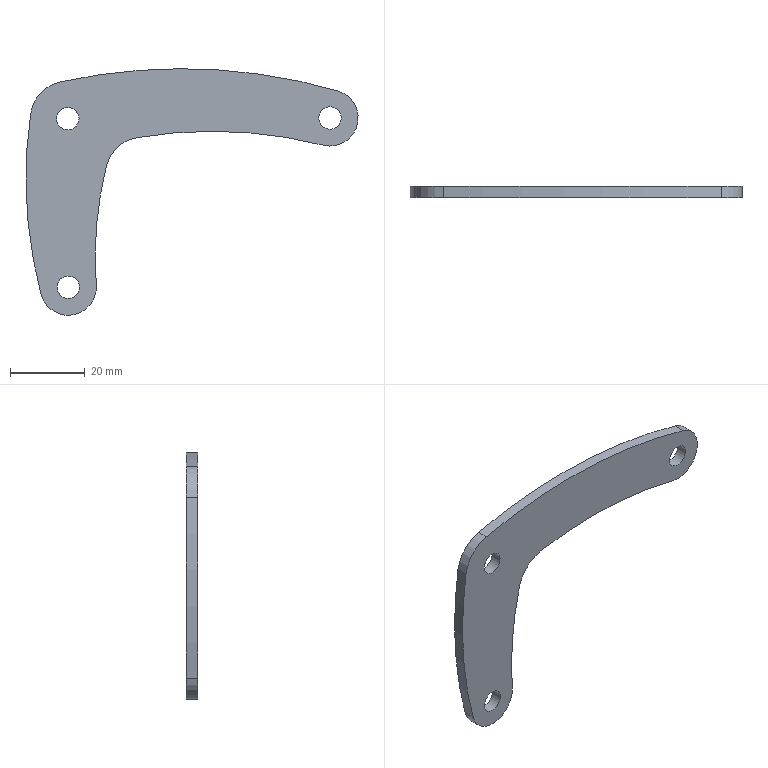Component | NX | LINK_2_3 | 1 solid | 13 faces | box 88.67 x 3 x 65.83 mm | volume 6437 mm3 | cylinder 11 | plane 2 | commonest cylinder face diameters 6 x3 240 x2 20 x2 15 x2 300 x1 200 x1
STEP:
#1=CARTESIAN_POINT('',(0.,0.,0.));
#2=DIRECTION('',(0.,0.,1.));
#3=DIRECTION('',(1.,0.,0.));
#4=AXIS2_PLACEMENT_3D('',#1,#2,#3);
#5=CARTESIAN_POINT('',(-172.247,90.,70.568));
#6=VERTEX_POINT('',#5);
#7=CARTESIAN_POINT('',(-175.02,90.,118.956));
#8=VERTEX_POINT('',#7);
#9=CARTESIAN_POINT('',(-56.298,90.,101.486));
#10=DIRECTION('',(0.,1.,0.));
#11=DIRECTION('',(-1.,0.,-0.002813));
#12=AXIS2_PLACEMENT_3D('',#9,#10,#11);
#13=CIRCLE('',#12,120.);
#14=CARTESIAN_POINT('',(-56.298,93.,101.486));
#15=DIRECTION('',(0.,-1.,0.));
#16=DIRECTION('',(-0.002813,0.,1.));
#17=AXIS2_PLACEMENT_3D('',#14,#15,#16);
#18=CYLINDRICAL_SURFACE('',#17,120.);
#19=CARTESIAN_POINT('',(7.854,3.));
#20=DIRECTION('',(-1.,0.));
#21=VECTOR('',#20,1.);
#22=LINE('',#19,#21);
#23=(GEOMETRIC_REPRESENTATION_CONTEXT(2)PARAMETRIC_REPRESENTATION_CONTEXT()REPRESENTATION_CONTEXT('',''));
#24=DEFINITIONAL_REPRESENTATION('',(#22),#23);
#25=PCURVE('',#18,#24);
#26=CARTESIAN_POINT('',(-110.713,90.,109.493));
#27=DIRECTION('',(0.,1.,0.));
#28=DIRECTION('',(0.002813,0.,-1.));
#29=AXIS2_PLACEMENT_3D('',#26,#27,#28);
#30=PLANE('',#29);
#31=CARTESIAN_POINT('',(8.16,-54.391));
#32=DIRECTION('',(0.,1.));
#33=AXIS2_PLACEMENT_2D('',#31,#32);
#34=CIRCLE('',#33,120.);
#35=(GEOMETRIC_REPRESENTATION_CONTEXT(2)PARAMETRIC_REPRESENTATION_CONTEXT()REPRESENTATION_CONTEXT('',''));
#36=DEFINITIONAL_REPRESENTATION('',(#34),#35);
#37=PCURVE('',#30,#36);
#38=SURFACE_CURVE('',#13,(#25,#37),.PCURVE_S1.);
#39=EDGE_CURVE('',#6,#8,#38,.T.);
#40=ORIENTED_EDGE('',*,*,#39,.T.);
#41=CARTESIAN_POINT('',(-175.02,93.,118.956));
#42=VERTEX_POINT('',#41);
#43=CARTESIAN_POINT('',(-175.02,93.,118.956));
#44=DIRECTION('',(0.,-1.,0.));
#45=VECTOR('',#44,1.);
#46=LINE('',#43,#45);
#47=CARTESIAN_POINT('',(1.422,0.));
#48=DIRECTION('',(0.,1.));
#49=VECTOR('',#48,1.);
#50=LINE('',#47,#49);
#51=(GEOMETRIC_REPRESENTATION_CONTEXT(2)PARAMETRIC_REPRESENTATION_CONTEXT()REPRESENTATION_CONTEXT('',''));
#52=DEFINITIONAL_REPRESENTATION('',(#50),#51);
#53=PCURVE('',#18,#52);
#54=CARTESIAN_POINT('',(-165.127,93.,117.5));
#55=DIRECTION('',(0.,-1.,0.));
#56=DIRECTION('',(-0.002813,0.,1.));
#57=AXIS2_PLACEMENT_3D('',#54,#55,#56);
#58=CYLINDRICAL_SURFACE('',#57,10.);
#59=CARTESIAN_POINT('',(1.422,0.));
#60=DIRECTION('',(0.,1.));
#61=VECTOR('',#60,1.);
#62=LINE('',#59,#61);
#63=(GEOMETRIC_REPRESENTATION_CONTEXT(2)PARAMETRIC_REPRESENTATION_CONTEXT()REPRESENTATION_CONTEXT('',''));
#64=DEFINITIONAL_REPRESENTATION('',(#62),#63);
#65=PCURVE('',#58,#64);
#66=SURFACE_CURVE('',#46,(#53,#65),.PCURVE_S1.);
#67=EDGE_CURVE('',#42,#8,#66,.T.);
#68=ORIENTED_EDGE('',*,*,#67,.F.);
#69=CARTESIAN_POINT('',(-172.247,93.,70.568));
#70=VERTEX_POINT('',#69);
#71=CARTESIAN_POINT('',(-56.298,93.,101.486));
#72=DIRECTION('',(0.,1.,0.));
#73=DIRECTION('',(-1.,0.,-0.002813));
#74=AXIS2_PLACEMENT_3D('',#71,#72,#73);
#75=CIRCLE('',#74,120.);
#76=CARTESIAN_POINT('',(7.854,0.));
#77=DIRECTION('',(-1.,0.));
#78=VECTOR('',#77,1.);
#79=LINE('',#76,#78);
#80=(GEOMETRIC_REPRESENTATION_CONTEXT(2)PARAMETRIC_REPRESENTATION_CONTEXT()REPRESENTATION_CONTEXT('',''));
#81=DEFINITIONAL_REPRESENTATION('',(#79),#80);
#82=PCURVE('',#18,#81);
#83=CARTESIAN_POINT('',(-110.713,93.,109.493));
#84=DIRECTION('',(0.,1.,0.));
#85=DIRECTION('',(0.002813,0.,-1.));
#86=AXIS2_PLACEMENT_3D('',#83,#84,#85);
#87=PLANE('',#86);
#88=CARTESIAN_POINT('',(8.16,-54.391));
#89=DIRECTION('',(0.,1.));
#90=AXIS2_PLACEMENT_2D('',#88,#89);
#91=CIRCLE('',#90,120.);
#92=(GEOMETRIC_REPRESENTATION_CONTEXT(2)PARAMETRIC_REPRESENTATION_CONTEXT()REPRESENTATION_CONTEXT('',''));
#93=DEFINITIONAL_REPRESENTATION('',(#91),#92);
#94=PCURVE('',#87,#93);
#95=SURFACE_CURVE('',#75,(#82,#94),.PCURVE_S1.);
#96=EDGE_CURVE('',#70,#42,#95,.T.);
#97=ORIENTED_EDGE('',*,*,#96,.F.);
#98=CARTESIAN_POINT('',(-172.247,93.,70.568));
#99=DIRECTION('',(0.,-1.,0.));
#100=VECTOR('',#99,1.);
#101=LINE('',#98,#100);
#102=CARTESIAN_POINT('',(1.829,0.));
#103=DIRECTION('',(0.,1.));
#104=VECTOR('',#103,1.);
#105=LINE('',#102,#104);
#106=(GEOMETRIC_REPRESENTATION_CONTEXT(2)PARAMETRIC_REPRESENTATION_CONTEXT()REPRESENTATION_CONTEXT('',''));
#107=DEFINITIONAL_REPRESENTATION('',(#105),#106);
#108=PCURVE('',#18,#107);
#109=CARTESIAN_POINT('',(-165.,93.,72.5));
#110=DIRECTION('',(0.,-1.,0.));
#111=DIRECTION('',(-0.002813,0.,1.));
#112=AXIS2_PLACEMENT_3D('',#109,#110,#111);
#113=CYLINDRICAL_SURFACE('',#112,7.5);
#114=CARTESIAN_POINT('',(1.829,0.));
#115=DIRECTION('',(0.,1.));
#116=VECTOR('',#115,1.);
#117=LINE('',#114,#116);
#118=(GEOMETRIC_REPRESENTATION_CONTEXT(2)PARAMETRIC_REPRESENTATION_CONTEXT()REPRESENTATION_CONTEXT('',''));
#119=DEFINITIONAL_REPRESENTATION('',(#117),#118);
#120=PCURVE('',#113,#119);
#121=SURFACE_CURVE('',#101,(#108,#120),.PCURVE_S1.);
#122=EDGE_CURVE('',#70,#6,#121,.T.);
#123=ORIENTED_EDGE('',*,*,#122,.T.);
#124=EDGE_LOOP('',(#40,#68,#97,#123));
#125=FACE_BOUND('',#124,.T.);
#126=ADVANCED_FACE('',(#125),#18,.T.);
#127=CARTESIAN_POINT('',(-167.294,90.,127.262));
#128=VERTEX_POINT('',#127);
#129=CARTESIAN_POINT('',(-165.127,90.,117.5));
#130=DIRECTION('',(0.,1.,0.));
#131=DIRECTION('',(-1.,0.,-0.002813));
#132=AXIS2_PLACEMENT_3D('',#129,#130,#131);
#133=CIRCLE('',#132,10.);
#134=CARTESIAN_POINT('',(1.571,3.));
#135=DIRECTION('',(-1.,0.));
#136=VECTOR('',#135,1.);
#137=LINE('',#134,#136);
#138=(GEOMETRIC_REPRESENTATION_CONTEXT(2)PARAMETRIC_REPRESENTATION_CONTEXT()REPRESENTATION_CONTEXT('',''));
#139=DEFINITIONAL_REPRESENTATION('',(#137),#138);
#140=PCURVE('',#58,#139);
#141=CARTESIAN_POINT('',(-8.16,54.391));
#142=DIRECTION('',(0.,1.));
#143=AXIS2_PLACEMENT_2D('',#141,#142);
#144=CIRCLE('',#143,10.);
#145=(GEOMETRIC_REPRESENTATION_CONTEXT(2)PARAMETRIC_REPRESENTATION_CONTEXT()REPRESENTATION_CONTEXT('',''));
#146=DEFINITIONAL_REPRESENTATION('',(#144),#145);
#147=PCURVE('',#30,#146);
#148=SURFACE_CURVE('',#133,(#140,#147),.PCURVE_S1.);
#149=EDGE_CURVE('',#8,#128,#148,.T.);
#150=ORIENTED_EDGE('',*,*,#149,.T.);
#151=CARTESIAN_POINT('',(-167.294,93.,127.262));
#152=VERTEX_POINT('',#151);
#153=CARTESIAN_POINT('',(-167.294,93.,127.262));
#154=DIRECTION('',(0.,-1.,0.));
#155=VECTOR('',#154,1.);
#156=LINE('',#153,#155);
#157=CARTESIAN_POINT('',(0.2156,0.));
#158=DIRECTION('',(0.,1.));
#159=VECTOR('',#158,1.);
#160=LINE('',#157,#159);
#161=(GEOMETRIC_REPRESENTATION_CONTEXT(2)PARAMETRIC_REPRESENTATION_CONTEXT()REPRESENTATION_CONTEXT('',''));
#162=DEFINITIONAL_REPRESENTATION('',(#160),#161);
#163=PCURVE('',#58,#162);
#164=CARTESIAN_POINT('',(-134.787,93.,-19.173));
#165=DIRECTION('',(0.,-1.,0.));
#166=DIRECTION('',(-0.002813,0.,1.));
#167=AXIS2_PLACEMENT_3D('',#164,#165,#166);
#168=CYLINDRICAL_SURFACE('',#167,150.);
#169=CARTESIAN_POINT('',(6.499,0.));
#170=DIRECTION('',(0.,1.));
#171=VECTOR('',#170,1.);
#172=LINE('',#169,#171);
#173=(GEOMETRIC_REPRESENTATION_CONTEXT(2)PARAMETRIC_REPRESENTATION_CONTEXT()REPRESENTATION_CONTEXT('',''));
#174=DEFINITIONAL_REPRESENTATION('',(#172),#173);
#175=PCURVE('',#168,#174);
#176=SURFACE_CURVE('',#156,(#163,#175),.PCURVE_S1.);
#177=EDGE_CURVE('',#152,#128,#176,.T.);
#178=ORIENTED_EDGE('',*,*,#177,.F.);
#179=CARTESIAN_POINT('',(-165.127,93.,117.5));
#180=DIRECTION('',(0.,1.,0.));
#181=DIRECTION('',(-1.,0.,-0.002813));
#182=AXIS2_PLACEMENT_3D('',#179,#180,#181);
#183=CIRCLE('',#182,10.);
#184=CARTESIAN_POINT('',(1.571,0.));
#185=DIRECTION('',(-1.,0.));
#186=VECTOR('',#185,1.);
#187=LINE('',#184,#186);
#188=(GEOMETRIC_REPRESENTATION_CONTEXT(2)PARAMETRIC_REPRESENTATION_CONTEXT()REPRESENTATION_CONTEXT('',''));
#189=DEFINITIONAL_REPRESENTATION('',(#187),#188);
#190=PCURVE('',#58,#189);
#191=CARTESIAN_POINT('',(-8.16,54.391));
#192=DIRECTION('',(0.,1.));
#193=AXIS2_PLACEMENT_2D('',#191,#192);
#194=CIRCLE('',#193,10.);
#195=(GEOMETRIC_REPRESENTATION_CONTEXT(2)PARAMETRIC_REPRESENTATION_CONTEXT()REPRESENTATION_CONTEXT('',''));
#196=DEFINITIONAL_REPRESENTATION('',(#194),#195);
#197=PCURVE('',#87,#196);
#198=SURFACE_CURVE('',#183,(#190,#197),.PCURVE_S1.);
#199=EDGE_CURVE('',#42,#152,#198,.T.);
#200=ORIENTED_EDGE('',*,*,#199,.F.);
#201=ORIENTED_EDGE('',*,*,#67,.T.);
#202=EDGE_LOOP('',(#150,#178,#200,#201));
#203=FACE_BOUND('',#202,.T.);
#204=ADVANCED_FACE('',(#203),#58,.T.);
#205=CARTESIAN_POINT('',(-93.04,90.,124.9));
#206=VERTEX_POINT('',#205);
#207=CARTESIAN_POINT('',(-134.787,90.,-19.173));
#208=DIRECTION('',(0.,1.,0.));
#209=DIRECTION('',(-1.,0.,-0.002813));
#210=AXIS2_PLACEMENT_3D('',#207,#208,#209);
#211=CIRCLE('',#210,150.);
#212=CARTESIAN_POINT('',(7.854,3.));
#213=DIRECTION('',(-1.,0.));
#214=VECTOR('',#213,1.);
#215=LINE('',#212,#214);
#216=(GEOMETRIC_REPRESENTATION_CONTEXT(2)PARAMETRIC_REPRESENTATION_CONTEXT()REPRESENTATION_CONTEXT('',''));
#217=DEFINITIONAL_REPRESENTATION('',(#215),#216);
#218=PCURVE('',#168,#217);
#219=CARTESIAN_POINT('',(128.598,24.436));
#220=DIRECTION('',(0.,1.));
#221=AXIS2_PLACEMENT_2D('',#219,#220);
#222=CIRCLE('',#221,150.);
#223=(GEOMETRIC_REPRESENTATION_CONTEXT(2)PARAMETRIC_REPRESENTATION_CONTEXT()REPRESENTATION_CONTEXT('',''));
#224=DEFINITIONAL_REPRESENTATION('',(#222),#223);
#225=PCURVE('',#30,#224);
#226=SURFACE_CURVE('',#211,(#218,#225),.PCURVE_S1.);
#227=EDGE_CURVE('',#128,#206,#226,.T.);
#228=ORIENTED_EDGE('',*,*,#227,.T.);
#229=CARTESIAN_POINT('',(-93.04,93.,124.9));
#230=VERTEX_POINT('',#229);
#231=CARTESIAN_POINT('',(-93.04,93.,124.9));
#232=DIRECTION('',(0.,-1.,0.));
#233=VECTOR('',#232,1.);
#234=LINE('',#231,#233);
#235=CARTESIAN_POINT('',(5.998,0.));
#236=DIRECTION('',(0.,1.));
#237=VECTOR('',#236,1.);
#238=LINE('',#235,#237);
#239=(GEOMETRIC_REPRESENTATION_CONTEXT(2)PARAMETRIC_REPRESENTATION_CONTEXT()REPRESENTATION_CONTEXT('',''));
#240=DEFINITIONAL_REPRESENTATION('',(#238),#239);
#241=PCURVE('',#168,#240);
#242=CARTESIAN_POINT('',(-95.127,93.,117.697));
#243=DIRECTION('',(0.,-1.,0.));
#244=DIRECTION('',(-0.002813,0.,1.));
#245=AXIS2_PLACEMENT_3D('',#242,#243,#244);
#246=CYLINDRICAL_SURFACE('',#245,7.5);
#247=CARTESIAN_POINT('',(5.998,0.));
#248=DIRECTION('',(0.,1.));
#249=VECTOR('',#248,1.);
#250=LINE('',#247,#249);
#251=(GEOMETRIC_REPRESENTATION_CONTEXT(2)PARAMETRIC_REPRESENTATION_CONTEXT()REPRESENTATION_CONTEXT('',''));
#252=DEFINITIONAL_REPRESENTATION('',(#250),#251);
#253=PCURVE('',#246,#252);
#254=SURFACE_CURVE('',#234,(#241,#253),.PCURVE_S1.);
#255=EDGE_CURVE('',#230,#206,#254,.T.);
#256=ORIENTED_EDGE('',*,*,#255,.F.);
#257=CARTESIAN_POINT('',(-134.787,93.,-19.173));
#258=DIRECTION('',(0.,1.,0.));
#259=DIRECTION('',(-1.,0.,-0.002813));
#260=AXIS2_PLACEMENT_3D('',#257,#258,#259);
#261=CIRCLE('',#260,150.);
#262=CARTESIAN_POINT('',(7.854,0.));
#263=DIRECTION('',(-1.,0.));
#264=VECTOR('',#263,1.);
#265=LINE('',#262,#264);
#266=(GEOMETRIC_REPRESENTATION_CONTEXT(2)PARAMETRIC_REPRESENTATION_CONTEXT()REPRESENTATION_CONTEXT('',''));
#267=DEFINITIONAL_REPRESENTATION('',(#265),#266);
#268=PCURVE('',#168,#267);
#269=CARTESIAN_POINT('',(128.598,24.436));
#270=DIRECTION('',(0.,1.));
#271=AXIS2_PLACEMENT_2D('',#269,#270);
#272=CIRCLE('',#271,150.);
#273=(GEOMETRIC_REPRESENTATION_CONTEXT(2)PARAMETRIC_REPRESENTATION_CONTEXT()REPRESENTATION_CONTEXT('',''));
#274=DEFINITIONAL_REPRESENTATION('',(#272),#273);
#275=PCURVE('',#87,#274);
#276=SURFACE_CURVE('',#261,(#268,#275),.PCURVE_S1.);
#277=EDGE_CURVE('',#152,#230,#276,.T.);
#278=ORIENTED_EDGE('',*,*,#277,.F.);
#279=ORIENTED_EDGE('',*,*,#177,.T.);
#280=EDGE_LOOP('',(#228,#256,#278,#279));
#281=FACE_BOUND('',#280,.T.);
#282=ADVANCED_FACE('',(#281),#168,.T.);
#283=CARTESIAN_POINT('',(-96.975,90.,110.428));
#284=VERTEX_POINT('',#283);
#285=CARTESIAN_POINT('',(-95.127,90.,117.697));
#286=DIRECTION('',(0.,1.,0.));
#287=DIRECTION('',(-1.,0.,-0.002813));
#288=AXIS2_PLACEMENT_3D('',#285,#286,#287);
#289=CIRCLE('',#288,7.5);
#290=CARTESIAN_POINT('',(7.854,3.));
#291=DIRECTION('',(-1.,0.));
#292=VECTOR('',#291,1.);
#293=LINE('',#290,#292);
#294=(GEOMETRIC_REPRESENTATION_CONTEXT(2)PARAMETRIC_REPRESENTATION_CONTEXT()REPRESENTATION_CONTEXT('',''));
#295=DEFINITIONAL_REPRESENTATION('',(#293),#294);
#296=PCURVE('',#246,#295);
#297=CARTESIAN_POINT('',(-8.16,-15.609));
#298=DIRECTION('',(-0.,1.));
#299=AXIS2_PLACEMENT_2D('',#297,#298);
#300=CIRCLE('',#299,7.5);
#301=(GEOMETRIC_REPRESENTATION_CONTEXT(2)PARAMETRIC_REPRESENTATION_CONTEXT()REPRESENTATION_CONTEXT('',''));
#302=DEFINITIONAL_REPRESENTATION('',(#300),#301);
#303=PCURVE('',#30,#302);
#304=SURFACE_CURVE('',#289,(#296,#303),.PCURVE_S1.);
#305=EDGE_CURVE('',#206,#284,#304,.T.);
#306=ORIENTED_EDGE('',*,*,#305,.T.);
#307=CARTESIAN_POINT('',(-96.975,93.,110.428));
#308=VERTEX_POINT('',#307);
#309=CARTESIAN_POINT('',(-96.975,93.,110.428));
#310=DIRECTION('',(0.,-1.,0.));
#311=VECTOR('',#310,1.);
#312=LINE('',#309,#311);
#313=CARTESIAN_POINT('',(2.89,0.));
#314=DIRECTION('',(0.,1.));
#315=VECTOR('',#314,1.);
#316=LINE('',#313,#315);
#317=(GEOMETRIC_REPRESENTATION_CONTEXT(2)PARAMETRIC_REPRESENTATION_CONTEXT()REPRESENTATION_CONTEXT('',''));
#318=DEFINITIONAL_REPRESENTATION('',(#316),#317);
#319=PCURVE('',#246,#318);
#320=CARTESIAN_POINT('',(-126.548,93.,-5.871));
#321=DIRECTION('',(0.,-1.,0.));
#322=DIRECTION('',(-0.002813,0.,1.));
#323=AXIS2_PLACEMENT_3D('',#320,#321,#322);
#324=CYLINDRICAL_SURFACE('',#323,120.);
#325=CARTESIAN_POINT('',(6.031,0.));
#326=DIRECTION('',(0.,1.));
#327=VECTOR('',#326,1.);
#328=LINE('',#325,#327);
#329=(GEOMETRIC_REPRESENTATION_CONTEXT(2)PARAMETRIC_REPRESENTATION_CONTEXT()REPRESENTATION_CONTEXT('',''));
#330=DEFINITIONAL_REPRESENTATION('',(#328),#329);
#331=PCURVE('',#324,#330);
#332=SURFACE_CURVE('',#312,(#319,#331),.PCURVE_S1.);
#333=EDGE_CURVE('',#308,#284,#332,.T.);
#334=ORIENTED_EDGE('',*,*,#333,.F.);
#335=CARTESIAN_POINT('',(-95.127,93.,117.697));
#336=DIRECTION('',(0.,1.,0.));
#337=DIRECTION('',(-1.,0.,-0.002813));
#338=AXIS2_PLACEMENT_3D('',#335,#336,#337);
#339=CIRCLE('',#338,7.5);
#340=CARTESIAN_POINT('',(7.854,0.));
#341=DIRECTION('',(-1.,0.));
#342=VECTOR('',#341,1.);
#343=LINE('',#340,#342);
#344=(GEOMETRIC_REPRESENTATION_CONTEXT(2)PARAMETRIC_REPRESENTATION_CONTEXT()REPRESENTATION_CONTEXT('',''));
#345=DEFINITIONAL_REPRESENTATION('',(#343),#344);
#346=PCURVE('',#246,#345);
#347=CARTESIAN_POINT('',(-8.16,-15.609));
#348=DIRECTION('',(-0.,1.));
#349=AXIS2_PLACEMENT_2D('',#347,#348);
#350=CIRCLE('',#349,7.5);
#351=(GEOMETRIC_REPRESENTATION_CONTEXT(2)PARAMETRIC_REPRESENTATION_CONTEXT()REPRESENTATION_CONTEXT('',''));
#352=DEFINITIONAL_REPRESENTATION('',(#350),#351);
#353=PCURVE('',#87,#352);
#354=SURFACE_CURVE('',#339,(#346,#353),.PCURVE_S1.);
#355=EDGE_CURVE('',#230,#308,#354,.T.);
#356=ORIENTED_EDGE('',*,*,#355,.F.);
#357=ORIENTED_EDGE('',*,*,#255,.T.);
#358=EDGE_LOOP('',(#306,#334,#356,#357));
#359=FACE_BOUND('',#358,.T.);
#360=ADVANCED_FACE('',(#359),#246,.T.);
#361=ORIENTED_EDGE('',*,*,#333,.F.);
#362=CARTESIAN_POINT('',(-146.77,93.,112.413));
#363=VERTEX_POINT('',#362);
#364=CARTESIAN_POINT('',(-126.548,93.,-5.871));
#365=DIRECTION('',(0.,-1.,0.));
#366=DIRECTION('',(-1.,0.,-0.002813));
#367=AXIS2_PLACEMENT_3D('',#364,#365,#366);
#368=CIRCLE('',#367,120.);
#369=CARTESIAN_POINT('',(1.571,0.));
#370=DIRECTION('',(1.,0.));
#371=VECTOR('',#370,1.);
#372=LINE('',#369,#371);
#373=(GEOMETRIC_REPRESENTATION_CONTEXT(2)PARAMETRIC_REPRESENTATION_CONTEXT()REPRESENTATION_CONTEXT('',''));
#374=DEFINITIONAL_REPRESENTATION('',(#372),#373);
#375=PCURVE('',#324,#374);
#376=CARTESIAN_POINT('',(115.319,136.16));
#377=CARTESIAN_POINT('',(323.165,136.16));
#378=CARTESIAN_POINT('',(219.242,-43.84));
#379=CARTESIAN_POINT('',(115.319,-223.84));
#380=CARTESIAN_POINT('',(11.396,-43.84));
#381=CARTESIAN_POINT('',(-92.527,136.16));
#382=CARTESIAN_POINT('',(115.319,136.16));
#383=(BOUNDED_CURVE()B_SPLINE_CURVE(2,(#376,#377,#378,#379,#380,#381,#382),.UNSPECIFIED.,.T.,.F.)B_SPLINE_CURVE_WITH_KNOTS((1,2,2,2,2,1),(-2.094,0.,2.094,4.189,6.283,8.378),.UNSPECIFIED.)CURVE()GEOMETRIC_REPRESENTATION_ITEM()RATIONAL_B_SPLINE_CURVE((1.,0.5,1.,0.5,1.,0.5,1.))REPRESENTATION_ITEM(''));
#384=(GEOMETRIC_REPRESENTATION_CONTEXT(2)PARAMETRIC_REPRESENTATION_CONTEXT()REPRESENTATION_CONTEXT('',''));
#385=DEFINITIONAL_REPRESENTATION('',(#383),#384);
#386=PCURVE('',#87,#385);
#387=SURFACE_CURVE('',#368,(#375,#386),.PCURVE_S1.);
#388=EDGE_CURVE('',#308,#363,#387,.T.);
#389=ORIENTED_EDGE('',*,*,#388,.T.);
#390=CARTESIAN_POINT('',(-146.77,90.,112.413));
#391=VERTEX_POINT('',#390);
#392=CARTESIAN_POINT('',(-146.77,93.,112.413));
#393=DIRECTION('',(0.,-1.,0.));
#394=VECTOR('',#393,1.);
#395=LINE('',#392,#394);
#396=CARTESIAN_POINT('',(6.45,0.));
#397=DIRECTION('',(0.,1.));
#398=VECTOR('',#397,1.);
#399=LINE('',#396,#398);
#400=(GEOMETRIC_REPRESENTATION_CONTEXT(2)PARAMETRIC_REPRESENTATION_CONTEXT()REPRESENTATION_CONTEXT('',''));
#401=DEFINITIONAL_REPRESENTATION('',(#399),#400);
#402=PCURVE('',#324,#401);
#403=CARTESIAN_POINT('',(-145.084,93.,102.556));
#404=DIRECTION('',(0.,-1.,0.));
#405=DIRECTION('',(-0.002813,0.,1.));
#406=AXIS2_PLACEMENT_3D('',#403,#404,#405);
#407=CYLINDRICAL_SURFACE('',#406,10.);
#408=CARTESIAN_POINT('',(0.1665,0.));
#409=DIRECTION('',(0.,1.));
#410=VECTOR('',#409,1.);
#411=LINE('',#408,#410);
#412=(GEOMETRIC_REPRESENTATION_CONTEXT(2)PARAMETRIC_REPRESENTATION_CONTEXT()REPRESENTATION_CONTEXT('',''));
#413=DEFINITIONAL_REPRESENTATION('',(#411),#412);
#414=PCURVE('',#407,#413);
#415=SURFACE_CURVE('',#395,(#402,#414),.PCURVE_S1.);
#416=EDGE_CURVE('',#363,#391,#415,.T.);
#417=ORIENTED_EDGE('',*,*,#416,.T.);
#418=CARTESIAN_POINT('',(-126.548,90.,-5.871));
#419=DIRECTION('',(0.,-1.,0.));
#420=DIRECTION('',(-1.,0.,-0.002813));
#421=AXIS2_PLACEMENT_3D('',#418,#419,#420);
#422=CIRCLE('',#421,120.);
#423=CARTESIAN_POINT('',(1.571,3.));
#424=DIRECTION('',(1.,0.));
#425=VECTOR('',#424,1.);
#426=LINE('',#423,#425);
#427=(GEOMETRIC_REPRESENTATION_CONTEXT(2)PARAMETRIC_REPRESENTATION_CONTEXT()REPRESENTATION_CONTEXT('',''));
#428=DEFINITIONAL_REPRESENTATION('',(#426),#427);
#429=PCURVE('',#324,#428);
#430=CARTESIAN_POINT('',(115.319,136.16));
#431=CARTESIAN_POINT('',(323.165,136.16));
#432=CARTESIAN_POINT('',(219.242,-43.84));
#433=CARTESIAN_POINT('',(115.319,-223.84));
#434=CARTESIAN_POINT('',(11.396,-43.84));
#435=CARTESIAN_POINT('',(-92.527,136.16));
#436=CARTESIAN_POINT('',(115.319,136.16));
#437=(BOUNDED_CURVE()B_SPLINE_CURVE(2,(#430,#431,#432,#433,#434,#435,#436),.UNSPECIFIED.,.T.,.F.)B_SPLINE_CURVE_WITH_KNOTS((1,2,2,2,2,1),(-2.094,0.,2.094,4.189,6.283,8.378),.UNSPECIFIED.)CURVE()GEOMETRIC_REPRESENTATION_ITEM()RATIONAL_B_SPLINE_CURVE((1.,0.5,1.,0.5,1.,0.5,1.))REPRESENTATION_ITEM(''));
#438=(GEOMETRIC_REPRESENTATION_CONTEXT(2)PARAMETRIC_REPRESENTATION_CONTEXT()REPRESENTATION_CONTEXT('',''));
#439=DEFINITIONAL_REPRESENTATION('',(#437),#438);
#440=PCURVE('',#30,#439);
#441=SURFACE_CURVE('',#422,(#429,#440),.PCURVE_S1.);
#442=EDGE_CURVE('',#284,#391,#441,.T.);
#443=ORIENTED_EDGE('',*,*,#442,.F.);
#444=EDGE_LOOP('',(#361,#389,#417,#443));
#445=FACE_BOUND('',#444,.F.);
#446=ADVANCED_FACE('',(#445),#324,.F.);
#447=ORIENTED_EDGE('',*,*,#416,.F.);
#448=CARTESIAN_POINT('',(-154.782,93.,104.996));
#449=VERTEX_POINT('',#448);
#450=CARTESIAN_POINT('',(-145.084,93.,102.556));
#451=DIRECTION('',(0.,-1.,0.));
#452=DIRECTION('',(-1.,0.,-0.002813));
#453=AXIS2_PLACEMENT_3D('',#450,#451,#452);
#454=CIRCLE('',#453,10.);
#455=CARTESIAN_POINT('',(-4.712,0.));
#456=DIRECTION('',(1.,0.));
#457=VECTOR('',#456,1.);
#458=LINE('',#455,#457);
#459=(GEOMETRIC_REPRESENTATION_CONTEXT(2)PARAMETRIC_REPRESENTATION_CONTEXT()REPRESENTATION_CONTEXT('',''));
#460=DEFINITIONAL_REPRESENTATION('',(#458),#459);
#461=PCURVE('',#407,#460);
#462=CARTESIAN_POINT('',(6.84,44.391));
#463=CARTESIAN_POINT('',(24.161,44.391));
#464=CARTESIAN_POINT('',(15.501,29.391));
#465=CARTESIAN_POINT('',(6.84,14.391));
#466=CARTESIAN_POINT('',(-1.82,29.391));
#467=CARTESIAN_POINT('',(-10.48,44.391));
#468=CARTESIAN_POINT('',(6.84,44.391));
#469=(BOUNDED_CURVE()B_SPLINE_CURVE(2,(#462,#463,#464,#465,#466,#467,#468),.UNSPECIFIED.,.T.,.F.)B_SPLINE_CURVE_WITH_KNOTS((1,2,2,2,2,1),(-2.094,0.,2.094,4.189,6.283,8.378),.UNSPECIFIED.)CURVE()GEOMETRIC_REPRESENTATION_ITEM()RATIONAL_B_SPLINE_CURVE((1.,0.5,1.,0.5,1.,0.5,1.))REPRESENTATION_ITEM(''));
#470=(GEOMETRIC_REPRESENTATION_CONTEXT(2)PARAMETRIC_REPRESENTATION_CONTEXT()REPRESENTATION_CONTEXT('',''));
#471=DEFINITIONAL_REPRESENTATION('',(#469),#470);
#472=PCURVE('',#87,#471);
#473=SURFACE_CURVE('',#454,(#461,#472),.PCURVE_S1.);
#474=EDGE_CURVE('',#363,#449,#473,.T.);
#475=ORIENTED_EDGE('',*,*,#474,.T.);
#476=CARTESIAN_POINT('',(-154.782,90.,104.996));
#477=VERTEX_POINT('',#476);
#478=CARTESIAN_POINT('',(-154.782,93.,104.996));
#479=DIRECTION('',(0.,-1.,0.));
#480=VECTOR('',#479,1.);
#481=LINE('',#478,#480);
#482=CARTESIAN_POINT('',(1.321,0.));
#483=DIRECTION('',(0.,1.));
#484=VECTOR('',#483,1.);
#485=LINE('',#482,#484);
#486=(GEOMETRIC_REPRESENTATION_CONTEXT(2)PARAMETRIC_REPRESENTATION_CONTEXT()REPRESENTATION_CONTEXT('',''));
#487=DEFINITIONAL_REPRESENTATION('',(#485),#486);
#488=PCURVE('',#407,#487);
#489=CARTESIAN_POINT('',(-57.805,93.,80.594));
#490=DIRECTION('',(0.,-1.,0.));
#491=DIRECTION('',(-0.002813,0.,1.));
#492=AXIS2_PLACEMENT_3D('',#489,#490,#491);
#493=CYLINDRICAL_SURFACE('',#492,100.);
#494=CARTESIAN_POINT('',(1.321,0.));
#495=DIRECTION('',(0.,1.));
#496=VECTOR('',#495,1.);
#497=LINE('',#494,#496);
#498=(GEOMETRIC_REPRESENTATION_CONTEXT(2)PARAMETRIC_REPRESENTATION_CONTEXT()REPRESENTATION_CONTEXT('',''));
#499=DEFINITIONAL_REPRESENTATION('',(#497),#498);
#500=PCURVE('',#493,#499);
#501=SURFACE_CURVE('',#481,(#488,#500),.PCURVE_S1.);
#502=EDGE_CURVE('',#449,#477,#501,.T.);
#503=ORIENTED_EDGE('',*,*,#502,.T.);
#504=CARTESIAN_POINT('',(-145.084,90.,102.556));
#505=DIRECTION('',(0.,-1.,0.));
#506=DIRECTION('',(-1.,0.,-0.002813));
#507=AXIS2_PLACEMENT_3D('',#504,#505,#506);
#508=CIRCLE('',#507,10.);
#509=CARTESIAN_POINT('',(-4.712,3.));
#510=DIRECTION('',(1.,0.));
#511=VECTOR('',#510,1.);
#512=LINE('',#509,#511);
#513=(GEOMETRIC_REPRESENTATION_CONTEXT(2)PARAMETRIC_REPRESENTATION_CONTEXT()REPRESENTATION_CONTEXT('',''));
#514=DEFINITIONAL_REPRESENTATION('',(#512),#513);
#515=PCURVE('',#407,#514);
#516=CARTESIAN_POINT('',(6.84,44.391));
#517=CARTESIAN_POINT('',(24.161,44.391));
#518=CARTESIAN_POINT('',(15.501,29.391));
#519=CARTESIAN_POINT('',(6.84,14.391));
#520=CARTESIAN_POINT('',(-1.82,29.391));
#521=CARTESIAN_POINT('',(-10.48,44.391));
#522=CARTESIAN_POINT('',(6.84,44.391));
#523=(BOUNDED_CURVE()B_SPLINE_CURVE(2,(#516,#517,#518,#519,#520,#521,#522),.UNSPECIFIED.,.T.,.F.)B_SPLINE_CURVE_WITH_KNOTS((1,2,2,2,2,1),(-2.094,0.,2.094,4.189,6.283,8.378),.UNSPECIFIED.)CURVE()GEOMETRIC_REPRESENTATION_ITEM()RATIONAL_B_SPLINE_CURVE((1.,0.5,1.,0.5,1.,0.5,1.))REPRESENTATION_ITEM(''));
#524=(GEOMETRIC_REPRESENTATION_CONTEXT(2)PARAMETRIC_REPRESENTATION_CONTEXT()REPRESENTATION_CONTEXT('',''));
#525=DEFINITIONAL_REPRESENTATION('',(#523),#524);
#526=PCURVE('',#30,#525);
#527=SURFACE_CURVE('',#508,(#515,#526),.PCURVE_S1.);
#528=EDGE_CURVE('',#391,#477,#527,.T.);
#529=ORIENTED_EDGE('',*,*,#528,.F.);
#530=EDGE_LOOP('',(#447,#475,#503,#529));
#531=FACE_BOUND('',#530,.F.);
#532=ADVANCED_FACE('',(#531),#407,.F.);
#533=ORIENTED_EDGE('',*,*,#502,.F.);
#534=CARTESIAN_POINT('',(-157.521,93.,73.065));
#535=VERTEX_POINT('',#534);
#536=CARTESIAN_POINT('',(-57.805,93.,80.594));
#537=DIRECTION('',(0.,-1.,0.));
#538=DIRECTION('',(-1.,0.,-0.002813));
#539=AXIS2_PLACEMENT_3D('',#536,#537,#538);
#540=CIRCLE('',#539,100.);
#541=CARTESIAN_POINT('',(-4.712,0.));
#542=DIRECTION('',(1.,0.));
#543=VECTOR('',#542,1.);
#544=LINE('',#541,#543);
#545=(GEOMETRIC_REPRESENTATION_CONTEXT(2)PARAMETRIC_REPRESENTATION_CONTEXT()REPRESENTATION_CONTEXT('',''));
#546=DEFINITIONAL_REPRESENTATION('',(#544),#545);
#547=PCURVE('',#493,#546);
#548=CARTESIAN_POINT('',(29.048,47.174));
#549=CARTESIAN_POINT('',(202.253,47.174));
#550=CARTESIAN_POINT('',(115.65,-102.826));
#551=CARTESIAN_POINT('',(29.048,-252.826));
#552=CARTESIAN_POINT('',(-57.555,-102.826));
#553=CARTESIAN_POINT('',(-144.158,47.174));
#554=CARTESIAN_POINT('',(29.048,47.174));
#555=(BOUNDED_CURVE()B_SPLINE_CURVE(2,(#548,#549,#550,#551,#552,#553,#554),.UNSPECIFIED.,.T.,.F.)B_SPLINE_CURVE_WITH_KNOTS((1,2,2,2,2,1),(-2.094,0.,2.094,4.189,6.283,8.378),.UNSPECIFIED.)CURVE()GEOMETRIC_REPRESENTATION_ITEM()RATIONAL_B_SPLINE_CURVE((1.,0.5,1.,0.5,1.,0.5,1.))REPRESENTATION_ITEM(''));
#556=(GEOMETRIC_REPRESENTATION_CONTEXT(2)PARAMETRIC_REPRESENTATION_CONTEXT()REPRESENTATION_CONTEXT('',''));
#557=DEFINITIONAL_REPRESENTATION('',(#555),#556);
#558=PCURVE('',#87,#557);
#559=SURFACE_CURVE('',#540,(#547,#558),.PCURVE_S1.);
#560=EDGE_CURVE('',#449,#535,#559,.T.);
#561=ORIENTED_EDGE('',*,*,#560,.T.);
#562=CARTESIAN_POINT('',(-157.521,90.,73.065));
#563=VERTEX_POINT('',#562);
#564=CARTESIAN_POINT('',(-157.521,93.,73.065));
#565=DIRECTION('',(0.,-1.,0.));
#566=VECTOR('',#565,1.);
#567=LINE('',#564,#566);
#568=CARTESIAN_POINT('',(1.643,0.));
#569=DIRECTION('',(0.,1.));
#570=VECTOR('',#569,1.);
#571=LINE('',#568,#570);
#572=(GEOMETRIC_REPRESENTATION_CONTEXT(2)PARAMETRIC_REPRESENTATION_CONTEXT()REPRESENTATION_CONTEXT('',''));
#573=DEFINITIONAL_REPRESENTATION('',(#571),#572);
#574=PCURVE('',#493,#573);
#575=CARTESIAN_POINT('',(4.785,0.));
#576=DIRECTION('',(0.,1.));
#577=VECTOR('',#576,1.);
#578=LINE('',#575,#577);
#579=(GEOMETRIC_REPRESENTATION_CONTEXT(2)PARAMETRIC_REPRESENTATION_CONTEXT()REPRESENTATION_CONTEXT('',''));
#580=DEFINITIONAL_REPRESENTATION('',(#578),#579);
#581=PCURVE('',#113,#580);
#582=SURFACE_CURVE('',#567,(#574,#581),.PCURVE_S1.);
#583=EDGE_CURVE('',#535,#563,#582,.T.);
#584=ORIENTED_EDGE('',*,*,#583,.T.);
#585=CARTESIAN_POINT('',(-57.805,90.,80.594));
#586=DIRECTION('',(0.,-1.,0.));
#587=DIRECTION('',(-1.,0.,-0.002813));
#588=AXIS2_PLACEMENT_3D('',#585,#586,#587);
#589=CIRCLE('',#588,100.);
#590=CARTESIAN_POINT('',(-4.712,3.));
#591=DIRECTION('',(1.,0.));
#592=VECTOR('',#591,1.);
#593=LINE('',#590,#592);
#594=(GEOMETRIC_REPRESENTATION_CONTEXT(2)PARAMETRIC_REPRESENTATION_CONTEXT()REPRESENTATION_CONTEXT('',''));
#595=DEFINITIONAL_REPRESENTATION('',(#593),#594);
#596=PCURVE('',#493,#595);
#597=CARTESIAN_POINT('',(29.048,47.174));
#598=CARTESIAN_POINT('',(202.253,47.174));
#599=CARTESIAN_POINT('',(115.65,-102.826));
#600=CARTESIAN_POINT('',(29.048,-252.826));
#601=CARTESIAN_POINT('',(-57.555,-102.826));
#602=CARTESIAN_POINT('',(-144.158,47.174));
#603=CARTESIAN_POINT('',(29.048,47.174));
#604=(BOUNDED_CURVE()B_SPLINE_CURVE(2,(#597,#598,#599,#600,#601,#602,#603),.UNSPECIFIED.,.T.,.F.)B_SPLINE_CURVE_WITH_KNOTS((1,2,2,2,2,1),(-2.094,0.,2.094,4.189,6.283,8.378),.UNSPECIFIED.)CURVE()GEOMETRIC_REPRESENTATION_ITEM()RATIONAL_B_SPLINE_CURVE((1.,0.5,1.,0.5,1.,0.5,1.))REPRESENTATION_ITEM(''));
#605=(GEOMETRIC_REPRESENTATION_CONTEXT(2)PARAMETRIC_REPRESENTATION_CONTEXT()REPRESENTATION_CONTEXT('',''));
#606=DEFINITIONAL_REPRESENTATION('',(#604),#605);
#607=PCURVE('',#30,#606);
#608=SURFACE_CURVE('',#589,(#596,#607),.PCURVE_S1.);
#609=EDGE_CURVE('',#477,#563,#608,.T.);
#610=ORIENTED_EDGE('',*,*,#609,.F.);
#611=EDGE_LOOP('',(#533,#561,#584,#610));
#612=FACE_BOUND('',#611,.F.);
#613=ADVANCED_FACE('',(#612),#493,.F.);
#614=CARTESIAN_POINT('',(-168.,93.,72.492));
#615=VERTEX_POINT('',#614);
#616=CARTESIAN_POINT('',(-165.,93.,72.5));
#617=DIRECTION('',(0.,1.,0.));
#618=DIRECTION('',(-1.,0.,-0.002813));
#619=AXIS2_PLACEMENT_3D('',#616,#617,#618);
#620=CIRCLE('',#619,3.);
#621=CARTESIAN_POINT('',(-165.,93.,72.5));
#622=DIRECTION('',(0.,-1.,0.));
#623=DIRECTION('',(-0.002813,0.,1.));
#624=AXIS2_PLACEMENT_3D('',#621,#622,#623);
#625=CYLINDRICAL_SURFACE('',#624,3.);
#626=CARTESIAN_POINT('',(7.854,0.));
#627=DIRECTION('',(-1.,0.));
#628=VECTOR('',#627,1.);
#629=LINE('',#626,#628);
#630=(GEOMETRIC_REPRESENTATION_CONTEXT(2)PARAMETRIC_REPRESENTATION_CONTEXT()REPRESENTATION_CONTEXT('',''));
#631=DEFINITIONAL_REPRESENTATION('',(#629),#630);
#632=PCURVE('',#625,#631);
#633=CARTESIAN_POINT('',(36.84,54.391));
#634=DIRECTION('',(-0.,1.));
#635=AXIS2_PLACEMENT_2D('',#633,#634);
#636=CIRCLE('',#635,3.);
#637=(GEOMETRIC_REPRESENTATION_CONTEXT(2)PARAMETRIC_REPRESENTATION_CONTEXT()REPRESENTATION_CONTEXT('',''));
#638=DEFINITIONAL_REPRESENTATION('',(#636),#637);
#639=PCURVE('',#87,#638);
#640=SURFACE_CURVE('',#620,(#632,#639),.PCURVE_S1.);
#641=EDGE_CURVE('',#615,#615,#640,.T.);
#642=ORIENTED_EDGE('',*,*,#641,.F.);
#643=CARTESIAN_POINT('',(-168.,90.,72.492));
#644=VERTEX_POINT('',#643);
#645=CARTESIAN_POINT('',(-168.,93.,72.492));
#646=CARTESIAN_POINT('',(-168.,90.,72.492));
#647=B_SPLINE_CURVE_WITH_KNOTS('',1,(#645,#646),.UNSPECIFIED.,.F.,.F.,(2,2),(0.,3.),.PIECEWISE_BEZIER_KNOTS.);
#648=CARTESIAN_POINT('',(7.854,0.));
#649=DIRECTION('',(0.,1.));
#650=VECTOR('',#649,1.);
#651=LINE('',#648,#650);
#652=(GEOMETRIC_REPRESENTATION_CONTEXT(2)PARAMETRIC_REPRESENTATION_CONTEXT()REPRESENTATION_CONTEXT('',''));
#653=DEFINITIONAL_REPRESENTATION('',(#651),#652);
#654=PCURVE('',#625,#653);
#655=CARTESIAN_POINT('',(1.571,0.));
#656=DIRECTION('',(0.,1.));
#657=VECTOR('',#656,1.);
#658=LINE('',#655,#657);
#659=(GEOMETRIC_REPRESENTATION_CONTEXT(2)PARAMETRIC_REPRESENTATION_CONTEXT()REPRESENTATION_CONTEXT('',''));
#660=DEFINITIONAL_REPRESENTATION('',(#658),#659);
#661=PCURVE('',#625,#660);
#662=SEAM_CURVE('',#647,(#654,#661),.PCURVE_S1.);
#663=EDGE_CURVE('',#615,#644,#662,.T.);
#664=ORIENTED_EDGE('',*,*,#663,.T.);
#665=CARTESIAN_POINT('',(-165.,90.,72.5));
#666=DIRECTION('',(0.,1.,0.));
#667=DIRECTION('',(-1.,0.,-0.002813));
#668=AXIS2_PLACEMENT_3D('',#665,#666,#667);
#669=CIRCLE('',#668,3.);
#670=CARTESIAN_POINT('',(7.854,3.));
#671=DIRECTION('',(-1.,0.));
#672=VECTOR('',#671,1.);
#673=LINE('',#670,#672);
#674=(GEOMETRIC_REPRESENTATION_CONTEXT(2)PARAMETRIC_REPRESENTATION_CONTEXT()REPRESENTATION_CONTEXT('',''));
#675=DEFINITIONAL_REPRESENTATION('',(#673),#674);
#676=PCURVE('',#625,#675);
#677=CARTESIAN_POINT('',(36.84,54.391));
#678=DIRECTION('',(-0.,1.));
#679=AXIS2_PLACEMENT_2D('',#677,#678);
#680=CIRCLE('',#679,3.);
#681=(GEOMETRIC_REPRESENTATION_CONTEXT(2)PARAMETRIC_REPRESENTATION_CONTEXT()REPRESENTATION_CONTEXT('',''));
#682=DEFINITIONAL_REPRESENTATION('',(#680),#681);
#683=PCURVE('',#30,#682);
#684=SURFACE_CURVE('',#669,(#676,#683),.PCURVE_S1.);
#685=EDGE_CURVE('',#644,#644,#684,.T.);
#686=ORIENTED_EDGE('',*,*,#685,.T.);
#687=ORIENTED_EDGE('',*,*,#663,.F.);
#688=EDGE_LOOP('',(#642,#664,#686,#687));
#689=FACE_BOUND('',#688,.F.);
#690=ADVANCED_FACE('',(#689),#625,.F.);
#691=CARTESIAN_POINT('',(-98.127,93.,117.688));
#692=VERTEX_POINT('',#691);
#693=CARTESIAN_POINT('',(-95.127,93.,117.697));
#694=DIRECTION('',(0.,1.,0.));
#695=DIRECTION('',(-1.,0.,-0.002813));
#696=AXIS2_PLACEMENT_3D('',#693,#694,#695);
#697=CIRCLE('',#696,3.);
#698=CARTESIAN_POINT('',(-95.127,93.,117.697));
#699=DIRECTION('',(0.,-1.,0.));
#700=DIRECTION('',(-0.002813,0.,1.));
#701=AXIS2_PLACEMENT_3D('',#698,#699,#700);
#702=CYLINDRICAL_SURFACE('',#701,3.);
#703=CARTESIAN_POINT('',(7.854,0.));
#704=DIRECTION('',(-1.,0.));
#705=VECTOR('',#704,1.);
#706=LINE('',#703,#705);
#707=(GEOMETRIC_REPRESENTATION_CONTEXT(2)PARAMETRIC_REPRESENTATION_CONTEXT()REPRESENTATION_CONTEXT('',''));
#708=DEFINITIONAL_REPRESENTATION('',(#706),#707);
#709=PCURVE('',#702,#708);
#710=CARTESIAN_POINT('',(-8.16,-15.609));
#711=DIRECTION('',(-0.,1.));
#712=AXIS2_PLACEMENT_2D('',#710,#711);
#713=CIRCLE('',#712,3.);
#714=(GEOMETRIC_REPRESENTATION_CONTEXT(2)PARAMETRIC_REPRESENTATION_CONTEXT()REPRESENTATION_CONTEXT('',''));
#715=DEFINITIONAL_REPRESENTATION('',(#713),#714);
#716=PCURVE('',#87,#715);
#717=SURFACE_CURVE('',#697,(#709,#716),.PCURVE_S1.);
#718=EDGE_CURVE('',#692,#692,#717,.T.);
#719=ORIENTED_EDGE('',*,*,#718,.F.);
#720=CARTESIAN_POINT('',(-98.127,90.,117.688));
#721=VERTEX_POINT('',#720);
#722=CARTESIAN_POINT('',(-98.127,93.,117.688));
#723=CARTESIAN_POINT('',(-98.127,90.,117.688));
#724=B_SPLINE_CURVE_WITH_KNOTS('',1,(#722,#723),.UNSPECIFIED.,.F.,.F.,(2,2),(0.,3.),.PIECEWISE_BEZIER_KNOTS.);
#725=CARTESIAN_POINT('',(7.854,0.));
#726=DIRECTION('',(0.,1.));
#727=VECTOR('',#726,1.);
#728=LINE('',#725,#727);
#729=(GEOMETRIC_REPRESENTATION_CONTEXT(2)PARAMETRIC_REPRESENTATION_CONTEXT()REPRESENTATION_CONTEXT('',''));
#730=DEFINITIONAL_REPRESENTATION('',(#728),#729);
#731=PCURVE('',#702,#730);
#732=CARTESIAN_POINT('',(1.571,0.));
#733=DIRECTION('',(0.,1.));
#734=VECTOR('',#733,1.);
#735=LINE('',#732,#734);
#736=(GEOMETRIC_REPRESENTATION_CONTEXT(2)PARAMETRIC_REPRESENTATION_CONTEXT()REPRESENTATION_CONTEXT('',''));
#737=DEFINITIONAL_REPRESENTATION('',(#735),#736);
#738=PCURVE('',#702,#737);
#739=SEAM_CURVE('',#724,(#731,#738),.PCURVE_S1.);
#740=EDGE_CURVE('',#692,#721,#739,.T.);
#741=ORIENTED_EDGE('',*,*,#740,.T.);
#742=CARTESIAN_POINT('',(-95.127,90.,117.697));
#743=DIRECTION('',(0.,1.,0.));
#744=DIRECTION('',(-1.,0.,-0.002813));
#745=AXIS2_PLACEMENT_3D('',#742,#743,#744);
#746=CIRCLE('',#745,3.);
#747=CARTESIAN_POINT('',(7.854,3.));
#748=DIRECTION('',(-1.,0.));
#749=VECTOR('',#748,1.);
#750=LINE('',#747,#749);
#751=(GEOMETRIC_REPRESENTATION_CONTEXT(2)PARAMETRIC_REPRESENTATION_CONTEXT()REPRESENTATION_CONTEXT('',''));
#752=DEFINITIONAL_REPRESENTATION('',(#750),#751);
#753=PCURVE('',#702,#752);
#754=CARTESIAN_POINT('',(-8.16,-15.609));
#755=DIRECTION('',(-0.,1.));
#756=AXIS2_PLACEMENT_2D('',#754,#755);
#757=CIRCLE('',#756,3.);
#758=(GEOMETRIC_REPRESENTATION_CONTEXT(2)PARAMETRIC_REPRESENTATION_CONTEXT()REPRESENTATION_CONTEXT('',''));
#759=DEFINITIONAL_REPRESENTATION('',(#757),#758);
#760=PCURVE('',#30,#759);
#761=SURFACE_CURVE('',#746,(#753,#760),.PCURVE_S1.);
#762=EDGE_CURVE('',#721,#721,#761,.T.);
#763=ORIENTED_EDGE('',*,*,#762,.T.);
#764=ORIENTED_EDGE('',*,*,#740,.F.);
#765=EDGE_LOOP('',(#719,#741,#763,#764));
#766=FACE_BOUND('',#765,.F.);
#767=ADVANCED_FACE('',(#766),#702,.F.);
#768=CARTESIAN_POINT('',(-165.,90.,72.5));
#769=DIRECTION('',(0.,1.,0.));
#770=DIRECTION('',(-1.,0.,-0.002813));
#771=AXIS2_PLACEMENT_3D('',#768,#769,#770);
#772=CIRCLE('',#771,7.5);
#773=CARTESIAN_POINT('',(7.854,3.));
#774=DIRECTION('',(-1.,0.));
#775=VECTOR('',#774,1.);
#776=LINE('',#773,#775);
#777=(GEOMETRIC_REPRESENTATION_CONTEXT(2)PARAMETRIC_REPRESENTATION_CONTEXT()REPRESENTATION_CONTEXT('',''));
#778=DEFINITIONAL_REPRESENTATION('',(#776),#777);
#779=PCURVE('',#113,#778);
#780=CARTESIAN_POINT('',(36.84,54.391));
#781=DIRECTION('',(-0.,1.));
#782=AXIS2_PLACEMENT_2D('',#780,#781);
#783=CIRCLE('',#782,7.5);
#784=(GEOMETRIC_REPRESENTATION_CONTEXT(2)PARAMETRIC_REPRESENTATION_CONTEXT()REPRESENTATION_CONTEXT('',''));
#785=DEFINITIONAL_REPRESENTATION('',(#783),#784);
#786=PCURVE('',#30,#785);
#787=SURFACE_CURVE('',#772,(#779,#786),.PCURVE_S1.);
#788=EDGE_CURVE('',#563,#6,#787,.T.);
#789=ORIENTED_EDGE('',*,*,#788,.T.);
#790=ORIENTED_EDGE('',*,*,#122,.F.);
#791=CARTESIAN_POINT('',(-165.,93.,72.5));
#792=DIRECTION('',(0.,1.,0.));
#793=DIRECTION('',(-1.,0.,-0.002813));
#794=AXIS2_PLACEMENT_3D('',#791,#792,#793);
#795=CIRCLE('',#794,7.5);
#796=CARTESIAN_POINT('',(7.854,0.));
#797=DIRECTION('',(-1.,0.));
#798=VECTOR('',#797,1.);
#799=LINE('',#796,#798);
#800=(GEOMETRIC_REPRESENTATION_CONTEXT(2)PARAMETRIC_REPRESENTATION_CONTEXT()REPRESENTATION_CONTEXT('',''));
#801=DEFINITIONAL_REPRESENTATION('',(#799),#800);
#802=PCURVE('',#113,#801);
#803=CARTESIAN_POINT('',(36.84,54.391));
#804=DIRECTION('',(-0.,1.));
#805=AXIS2_PLACEMENT_2D('',#803,#804);
#806=CIRCLE('',#805,7.5);
#807=(GEOMETRIC_REPRESENTATION_CONTEXT(2)PARAMETRIC_REPRESENTATION_CONTEXT()REPRESENTATION_CONTEXT('',''));
#808=DEFINITIONAL_REPRESENTATION('',(#806),#807);
#809=PCURVE('',#87,#808);
#810=SURFACE_CURVE('',#795,(#802,#809),.PCURVE_S1.);
#811=EDGE_CURVE('',#535,#70,#810,.T.);
#812=ORIENTED_EDGE('',*,*,#811,.F.);
#813=ORIENTED_EDGE('',*,*,#583,.T.);
#814=EDGE_LOOP('',(#789,#790,#812,#813));
#815=FACE_BOUND('',#814,.T.);
#816=ADVANCED_FACE('',(#815),#113,.T.);
#817=CARTESIAN_POINT('',(-168.127,93.,117.491));
#818=VERTEX_POINT('',#817);
#819=CARTESIAN_POINT('',(-165.127,93.,117.5));
#820=DIRECTION('',(0.,1.,0.));
#821=DIRECTION('',(-1.,0.,-0.002813));
#822=AXIS2_PLACEMENT_3D('',#819,#820,#821);
#823=CIRCLE('',#822,3.);
#824=CARTESIAN_POINT('',(-165.127,93.,117.5));
#825=DIRECTION('',(0.,-1.,0.));
#826=DIRECTION('',(-0.002813,0.,1.));
#827=AXIS2_PLACEMENT_3D('',#824,#825,#826);
#828=CYLINDRICAL_SURFACE('',#827,3.);
#829=CARTESIAN_POINT('',(7.854,0.));
#830=DIRECTION('',(-1.,0.));
#831=VECTOR('',#830,1.);
#832=LINE('',#829,#831);
#833=(GEOMETRIC_REPRESENTATION_CONTEXT(2)PARAMETRIC_REPRESENTATION_CONTEXT()REPRESENTATION_CONTEXT('',''));
#834=DEFINITIONAL_REPRESENTATION('',(#832),#833);
#835=PCURVE('',#828,#834);
#836=CARTESIAN_POINT('',(-8.16,54.391));
#837=DIRECTION('',(-0.,1.));
#838=AXIS2_PLACEMENT_2D('',#836,#837);
#839=CIRCLE('',#838,3.);
#840=(GEOMETRIC_REPRESENTATION_CONTEXT(2)PARAMETRIC_REPRESENTATION_CONTEXT()REPRESENTATION_CONTEXT('',''));
#841=DEFINITIONAL_REPRESENTATION('',(#839),#840);
#842=PCURVE('',#87,#841);
#843=SURFACE_CURVE('',#823,(#835,#842),.PCURVE_S1.);
#844=EDGE_CURVE('',#818,#818,#843,.T.);
#845=ORIENTED_EDGE('',*,*,#844,.F.);
#846=CARTESIAN_POINT('',(-168.127,90.,117.491));
#847=VERTEX_POINT('',#846);
#848=CARTESIAN_POINT('',(-168.127,93.,117.491));
#849=CARTESIAN_POINT('',(-168.127,90.,117.491));
#850=B_SPLINE_CURVE_WITH_KNOTS('',1,(#848,#849),.UNSPECIFIED.,.F.,.F.,(2,2),(0.,3.),.PIECEWISE_BEZIER_KNOTS.);
#851=CARTESIAN_POINT('',(7.854,0.));
#852=DIRECTION('',(0.,1.));
#853=VECTOR('',#852,1.);
#854=LINE('',#851,#853);
#855=(GEOMETRIC_REPRESENTATION_CONTEXT(2)PARAMETRIC_REPRESENTATION_CONTEXT()REPRESENTATION_CONTEXT('',''));
#856=DEFINITIONAL_REPRESENTATION('',(#854),#855);
#857=PCURVE('',#828,#856);
#858=CARTESIAN_POINT('',(1.571,0.));
#859=DIRECTION('',(0.,1.));
#860=VECTOR('',#859,1.);
#861=LINE('',#858,#860);
#862=(GEOMETRIC_REPRESENTATION_CONTEXT(2)PARAMETRIC_REPRESENTATION_CONTEXT()REPRESENTATION_CONTEXT('',''));
#863=DEFINITIONAL_REPRESENTATION('',(#861),#862);
#864=PCURVE('',#828,#863);
#865=SEAM_CURVE('',#850,(#857,#864),.PCURVE_S1.);
#866=EDGE_CURVE('',#818,#847,#865,.T.);
#867=ORIENTED_EDGE('',*,*,#866,.T.);
#868=CARTESIAN_POINT('',(-165.127,90.,117.5));
#869=DIRECTION('',(0.,1.,0.));
#870=DIRECTION('',(-1.,0.,-0.002813));
#871=AXIS2_PLACEMENT_3D('',#868,#869,#870);
#872=CIRCLE('',#871,3.);
#873=CARTESIAN_POINT('',(7.854,3.));
#874=DIRECTION('',(-1.,0.));
#875=VECTOR('',#874,1.);
#876=LINE('',#873,#875);
#877=(GEOMETRIC_REPRESENTATION_CONTEXT(2)PARAMETRIC_REPRESENTATION_CONTEXT()REPRESENTATION_CONTEXT('',''));
#878=DEFINITIONAL_REPRESENTATION('',(#876),#877);
#879=PCURVE('',#828,#878);
#880=CARTESIAN_POINT('',(-8.16,54.391));
#881=DIRECTION('',(-0.,1.));
#882=AXIS2_PLACEMENT_2D('',#880,#881);
#883=CIRCLE('',#882,3.);
#884=(GEOMETRIC_REPRESENTATION_CONTEXT(2)PARAMETRIC_REPRESENTATION_CONTEXT()REPRESENTATION_CONTEXT('',''));
#885=DEFINITIONAL_REPRESENTATION('',(#883),#884);
#886=PCURVE('',#30,#885);
#887=SURFACE_CURVE('',#872,(#879,#886),.PCURVE_S1.);
#888=EDGE_CURVE('',#847,#847,#887,.T.);
#889=ORIENTED_EDGE('',*,*,#888,.T.);
#890=ORIENTED_EDGE('',*,*,#866,.F.);
#891=EDGE_LOOP('',(#845,#867,#889,#890));
#892=FACE_BOUND('',#891,.F.);
#893=ADVANCED_FACE('',(#892),#828,.F.);
#894=ORIENTED_EDGE('',*,*,#96,.T.);
#895=ORIENTED_EDGE('',*,*,#199,.T.);
#896=ORIENTED_EDGE('',*,*,#277,.T.);
#897=ORIENTED_EDGE('',*,*,#355,.T.);
#898=ORIENTED_EDGE('',*,*,#388,.T.);
#899=ORIENTED_EDGE('',*,*,#474,.T.);
#900=ORIENTED_EDGE('',*,*,#560,.T.);
#901=ORIENTED_EDGE('',*,*,#811,.T.);
#902=EDGE_LOOP('',(#894,#895,#896,#897,#898,#899,#900,#901));
#903=FACE_BOUND('',#902,.T.);
#904=ORIENTED_EDGE('',*,*,#718,.F.);
#905=EDGE_LOOP('',(#904));
#906=FACE_BOUND('',#905,.T.);
#907=ORIENTED_EDGE('',*,*,#641,.F.);
#908=EDGE_LOOP('',(#907));
#909=FACE_BOUND('',#908,.T.);
#910=ORIENTED_EDGE('',*,*,#844,.F.);
#911=EDGE_LOOP('',(#910));
#912=FACE_BOUND('',#911,.T.);
#913=ADVANCED_FACE('',(#903,#906,#909,#912),#87,.T.);
#914=ORIENTED_EDGE('',*,*,#39,.F.);
#915=ORIENTED_EDGE('',*,*,#788,.F.);
#916=ORIENTED_EDGE('',*,*,#609,.F.);
#917=ORIENTED_EDGE('',*,*,#528,.F.);
#918=ORIENTED_EDGE('',*,*,#442,.F.);
#919=ORIENTED_EDGE('',*,*,#305,.F.);
#920=ORIENTED_EDGE('',*,*,#227,.F.);
#921=ORIENTED_EDGE('',*,*,#149,.F.);
#922=EDGE_LOOP('',(#914,#915,#916,#917,#918,#919,#920,#921));
#923=FACE_BOUND('',#922,.T.);
#924=ORIENTED_EDGE('',*,*,#762,.T.);
#925=EDGE_LOOP('',(#924));
#926=FACE_BOUND('',#925,.T.);
#927=ORIENTED_EDGE('',*,*,#685,.T.);
#928=EDGE_LOOP('',(#927));
#929=FACE_BOUND('',#928,.T.);
#930=ORIENTED_EDGE('',*,*,#888,.T.);
#931=EDGE_LOOP('',(#930));
#932=FACE_BOUND('',#931,.T.);
#933=ADVANCED_FACE('',(#923,#926,#929,#932),#30,.F.);
#934=CLOSED_SHELL('',(#126,#204,#282,#360,#446,#532,#613,#690,#767,#816,#893,#913,#933));
#935=MANIFOLD_SOLID_BREP('',#934);
#936=(LENGTH_UNIT()NAMED_UNIT(*)SI_UNIT(.MILLI.,.METRE.));
#937=UNCERTAINTY_MEASURE_WITH_UNIT(LENGTH_MEASURE(0.000002),#936,'','');
#938=(NAMED_UNIT(*)PLANE_ANGLE_UNIT()SI_UNIT($,.RADIAN.));
#939=(NAMED_UNIT(*)SI_UNIT($,.STERADIAN.)SOLID_ANGLE_UNIT());
#940=(GEOMETRIC_REPRESENTATION_CONTEXT(3)GLOBAL_UNCERTAINTY_ASSIGNED_CONTEXT((#937))GLOBAL_UNIT_ASSIGNED_CONTEXT((#936,#938,#939))REPRESENTATION_CONTEXT('',''));
#941=ADVANCED_BREP_SHAPE_REPRESENTATION('',(#4,#935),#940);